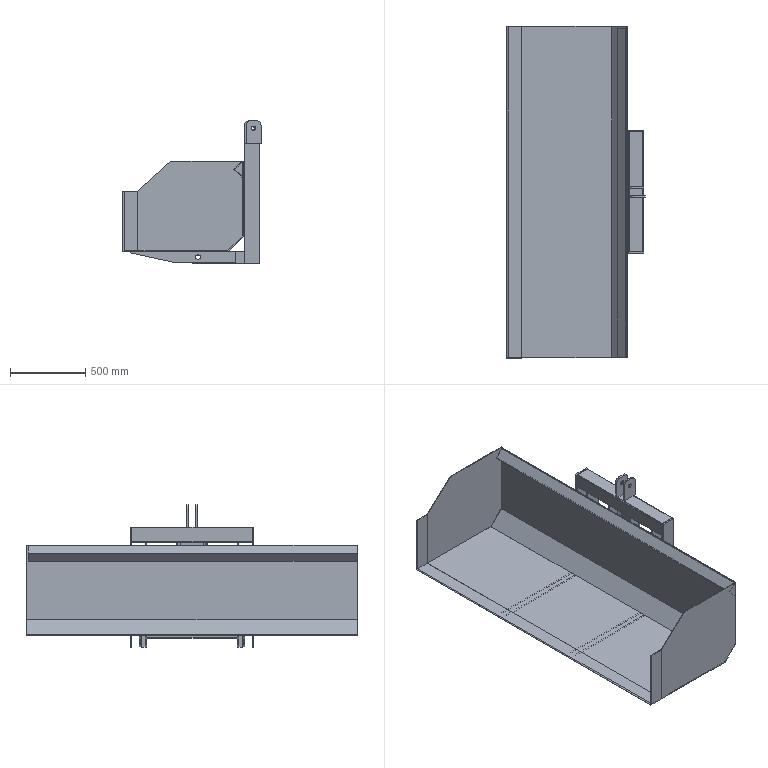Assembly | NX | mm | 20 component files | 20 solids | 181 faces | box 920 x 2210.07 x 950 mm | volume 31715430 mm3 | plane 153 | cylinder 28 | commonest cylinder face diameters 10 x8 31 x6 40 x4 60 x4 4 x4 28 x2
Bill of materials:
unnamed part 1 | 4 |  | Long thin flat bar. One edge is straight. On the other edge, about half the length runs parallel and then angles in, so the bar narrows to a pointed end. It has a single round through-hole.
unnamed part 2 | 2 |  | Flat rectangular tab plate. The two corners at one end are rounded and a single round through-hole sits near that end.
unnamed part 3 | 1 |  | Thin-walled C-shaped (channel) section of constant profile along its length. It has a web, two parallel flanges and rounded inside and outside bends.
unnamed part 4 | 1 |  | Straight hollow square tube with a thin wall and small outer corner radii. Both ends are cut square.
unnamed part 5 | 2 |  | Plain thin rectangular flat strip or plate with no holes or other features.
unnamed part 6 | 2 |  | Plain thin rectangular flat strip or plate with no holes or other features.
unnamed part 7 | 1 |  | Straight hollow square tube with a thin wall and small outer corner radii. Both ends are cut square.
unnamed part 8 | 1 |  | Thin sheet strip bent into a shallow U shape: a long flat base with a short upright flange at each end.
unnamed part 9 | 1 |  | Long angle section with a V-shaped profile. Two legs of about equal length meet at roughly 90 degrees, and the leg tips are rounded.
unnamed part 10 | 2 |  | Thin flat plate with an irregular polygon outline: a rectangle with two diagonally opposite corners chamfered, one larger than the other.
unnamed part 11 | 1 |  | Thin sheet profile with a wide flat leg and an upright leg. The two legs are joined by a short 45-degree angled segment instead of a sharp corner.
unnamed part 12 | 2 |  | Rectangular flat bar with a single round through-hole near one end.
Mates:
1. touch align | chapa_lateral 2 face | tubo 1 face
2. distance | tubo 1 face | chapa_lateral 2 face
3. touch align | tubo 1 face | chapa_lateral 2 face
4. touch align | perfil_u 1 | tubo 1 face
5. distance | perfil_u 1 | tubo 1 face
6. distance | tubo_inferior 1 | perfil_u 1
7. distance | tubo_inferior 1 | perfil_u 1
8. distance | tubo_inferior 1 | chapa_interna 2
9. distance | perfil_u 1 | chapa_lateral 2 face
10. distance | chapa_interna 2 | chapa_garfo 2
11. distance | chapa_garfo 2 | chapa_interna 2
12. distance | chapa_garfo 2 | chapa_interna 2
13. distance | chapa_garafa 2 | tubo 1 face
14. distance | chapa_garafa 2 | tubo 1 face
15. distance | chapa_garafa 2 | assembly datumplane
16. touch align | cacanba 2 | cacamba_2200 1
17. distance | cacamba_2200 1 | cacanba 2
18. distance | cacanba 2 | cacamba_2200 1
19. touch align | cantoneira 1 | cacanba 2
20. distance | cantoneira 1 | cacamba_2200 1
21. distance | cantoneira 1 | cacamba_2200 1
22. distance | chapa_fundo 4 | cacamba_2200 1
23. fix | assembly component
24. bond | chapa_fundo 4 component | assembly component
25. bond | chapa_fundo 3 component | assembly component
26. linear | assembly datumaxis | assembly cartesiancoordinatesystem | assembly cartesiancoordinatesystem
27. distance | chapa_fundo 3 | assembly datumplane
28. distance | chapa_fundo 2 | assembly datumplane
29. distance | chapa_fundo 2 | chapa_fundo 1
30. distance | plataforma_montada 1 datumplane | cavalete_plaforma 1 datumplane